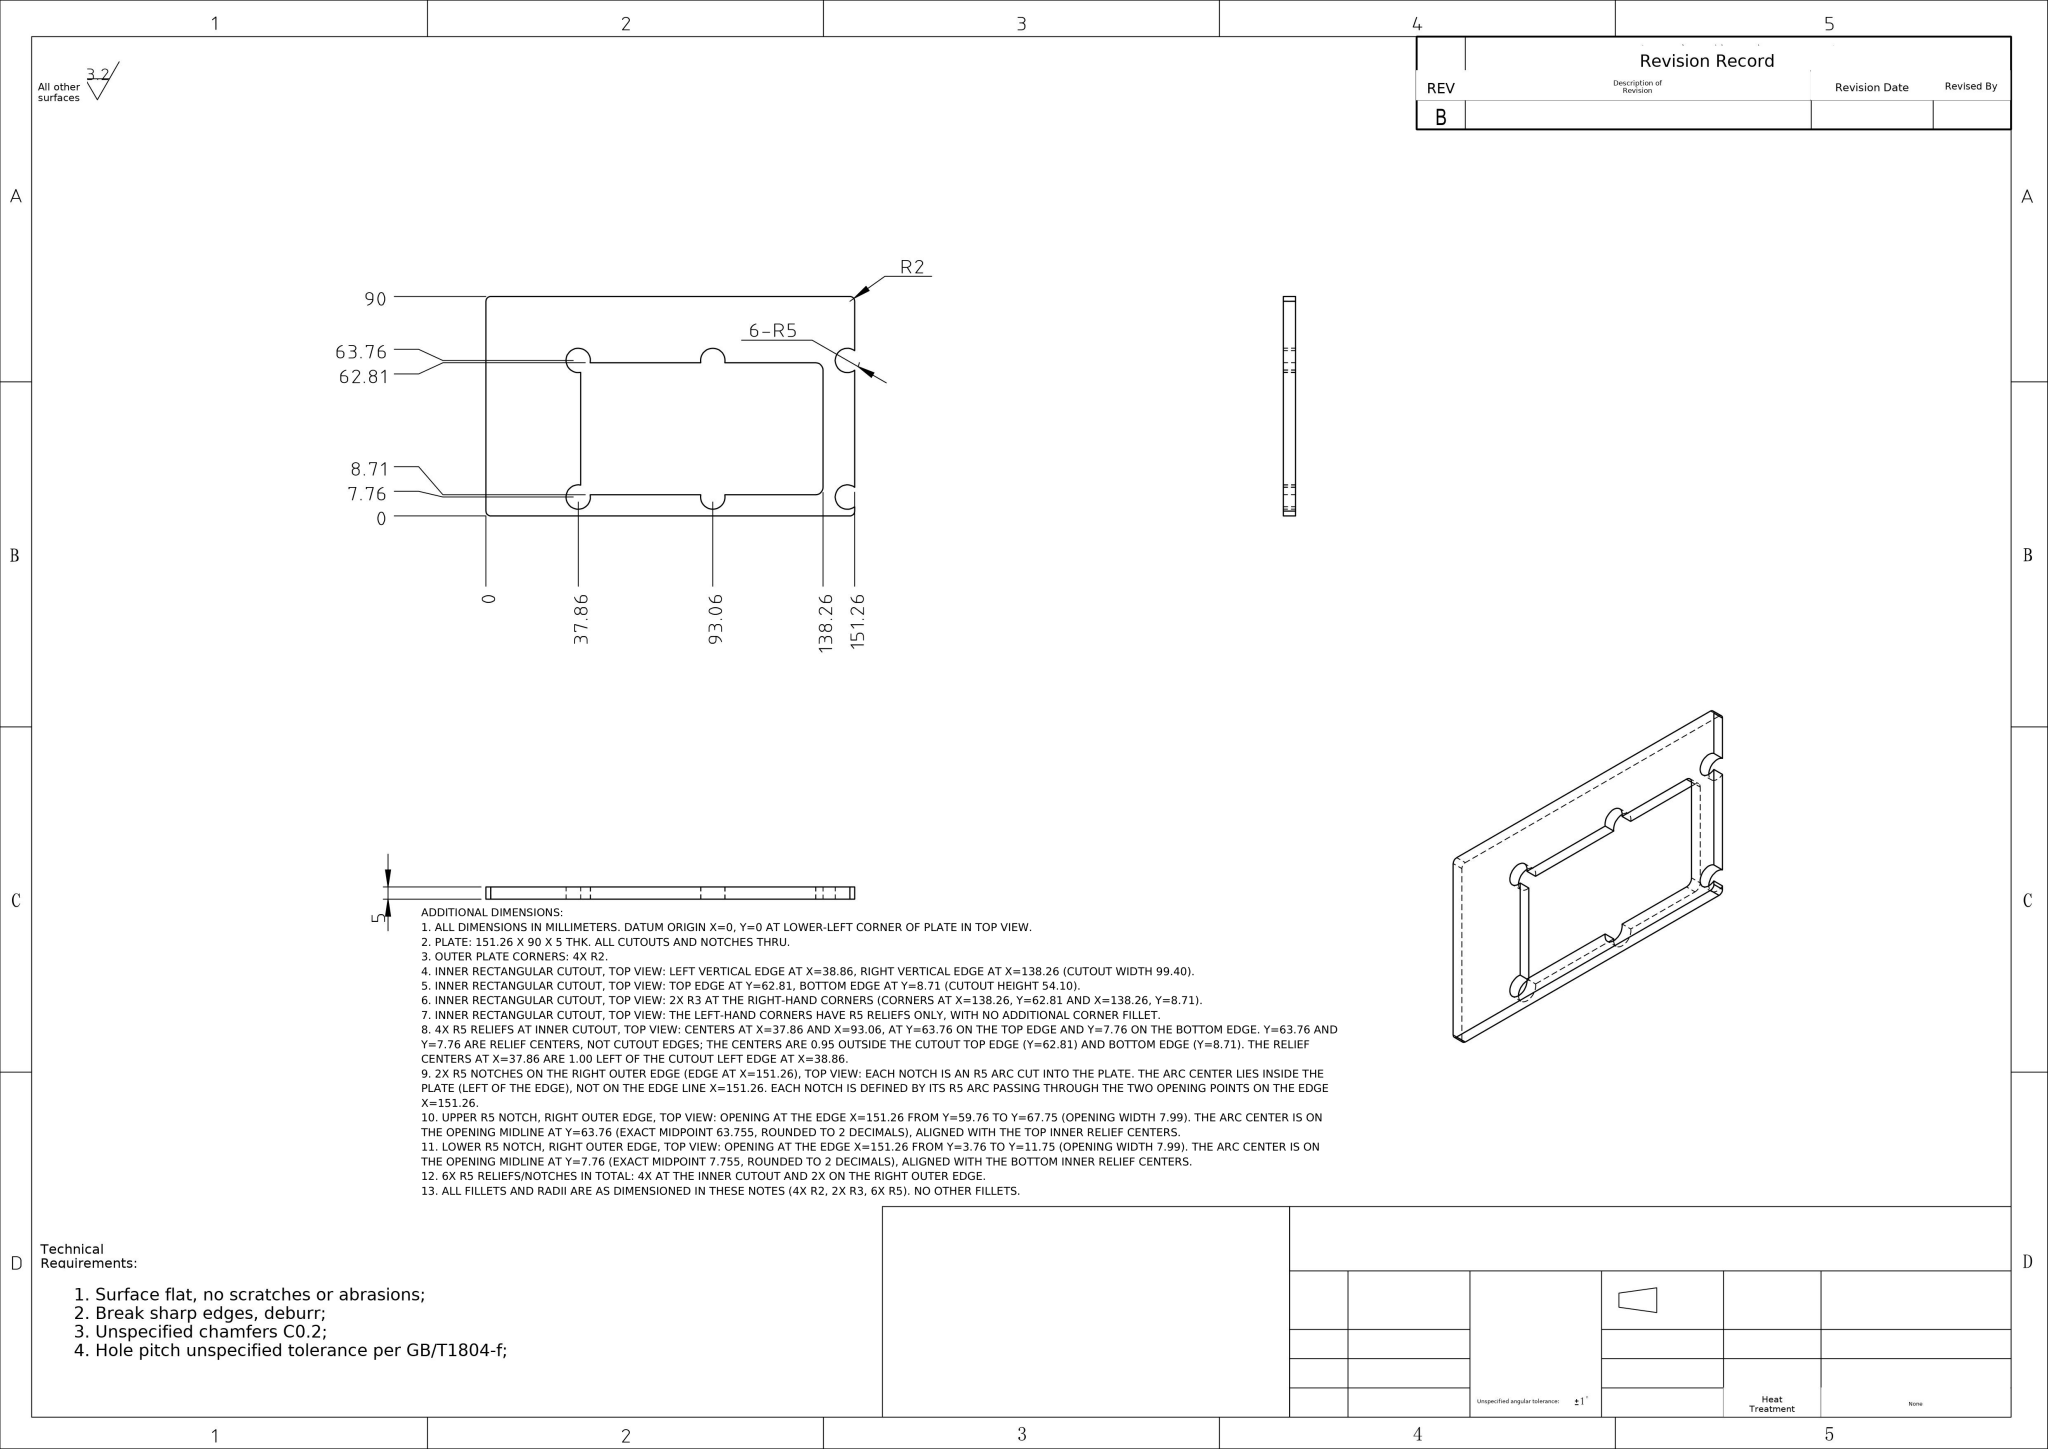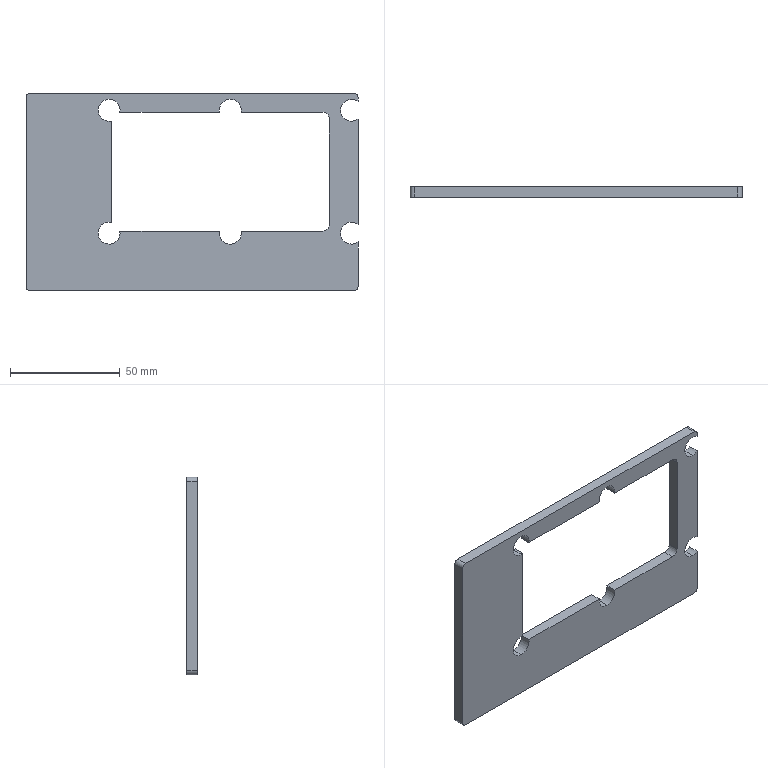Part | NX | mm | 1 solid | 35 faces | box 151.26 x 5 x 90 mm | volume 39342 mm3 | cylinder 21 | plane 14 | commonest cylinder face diameters 10 x15 4 x4 6 x2